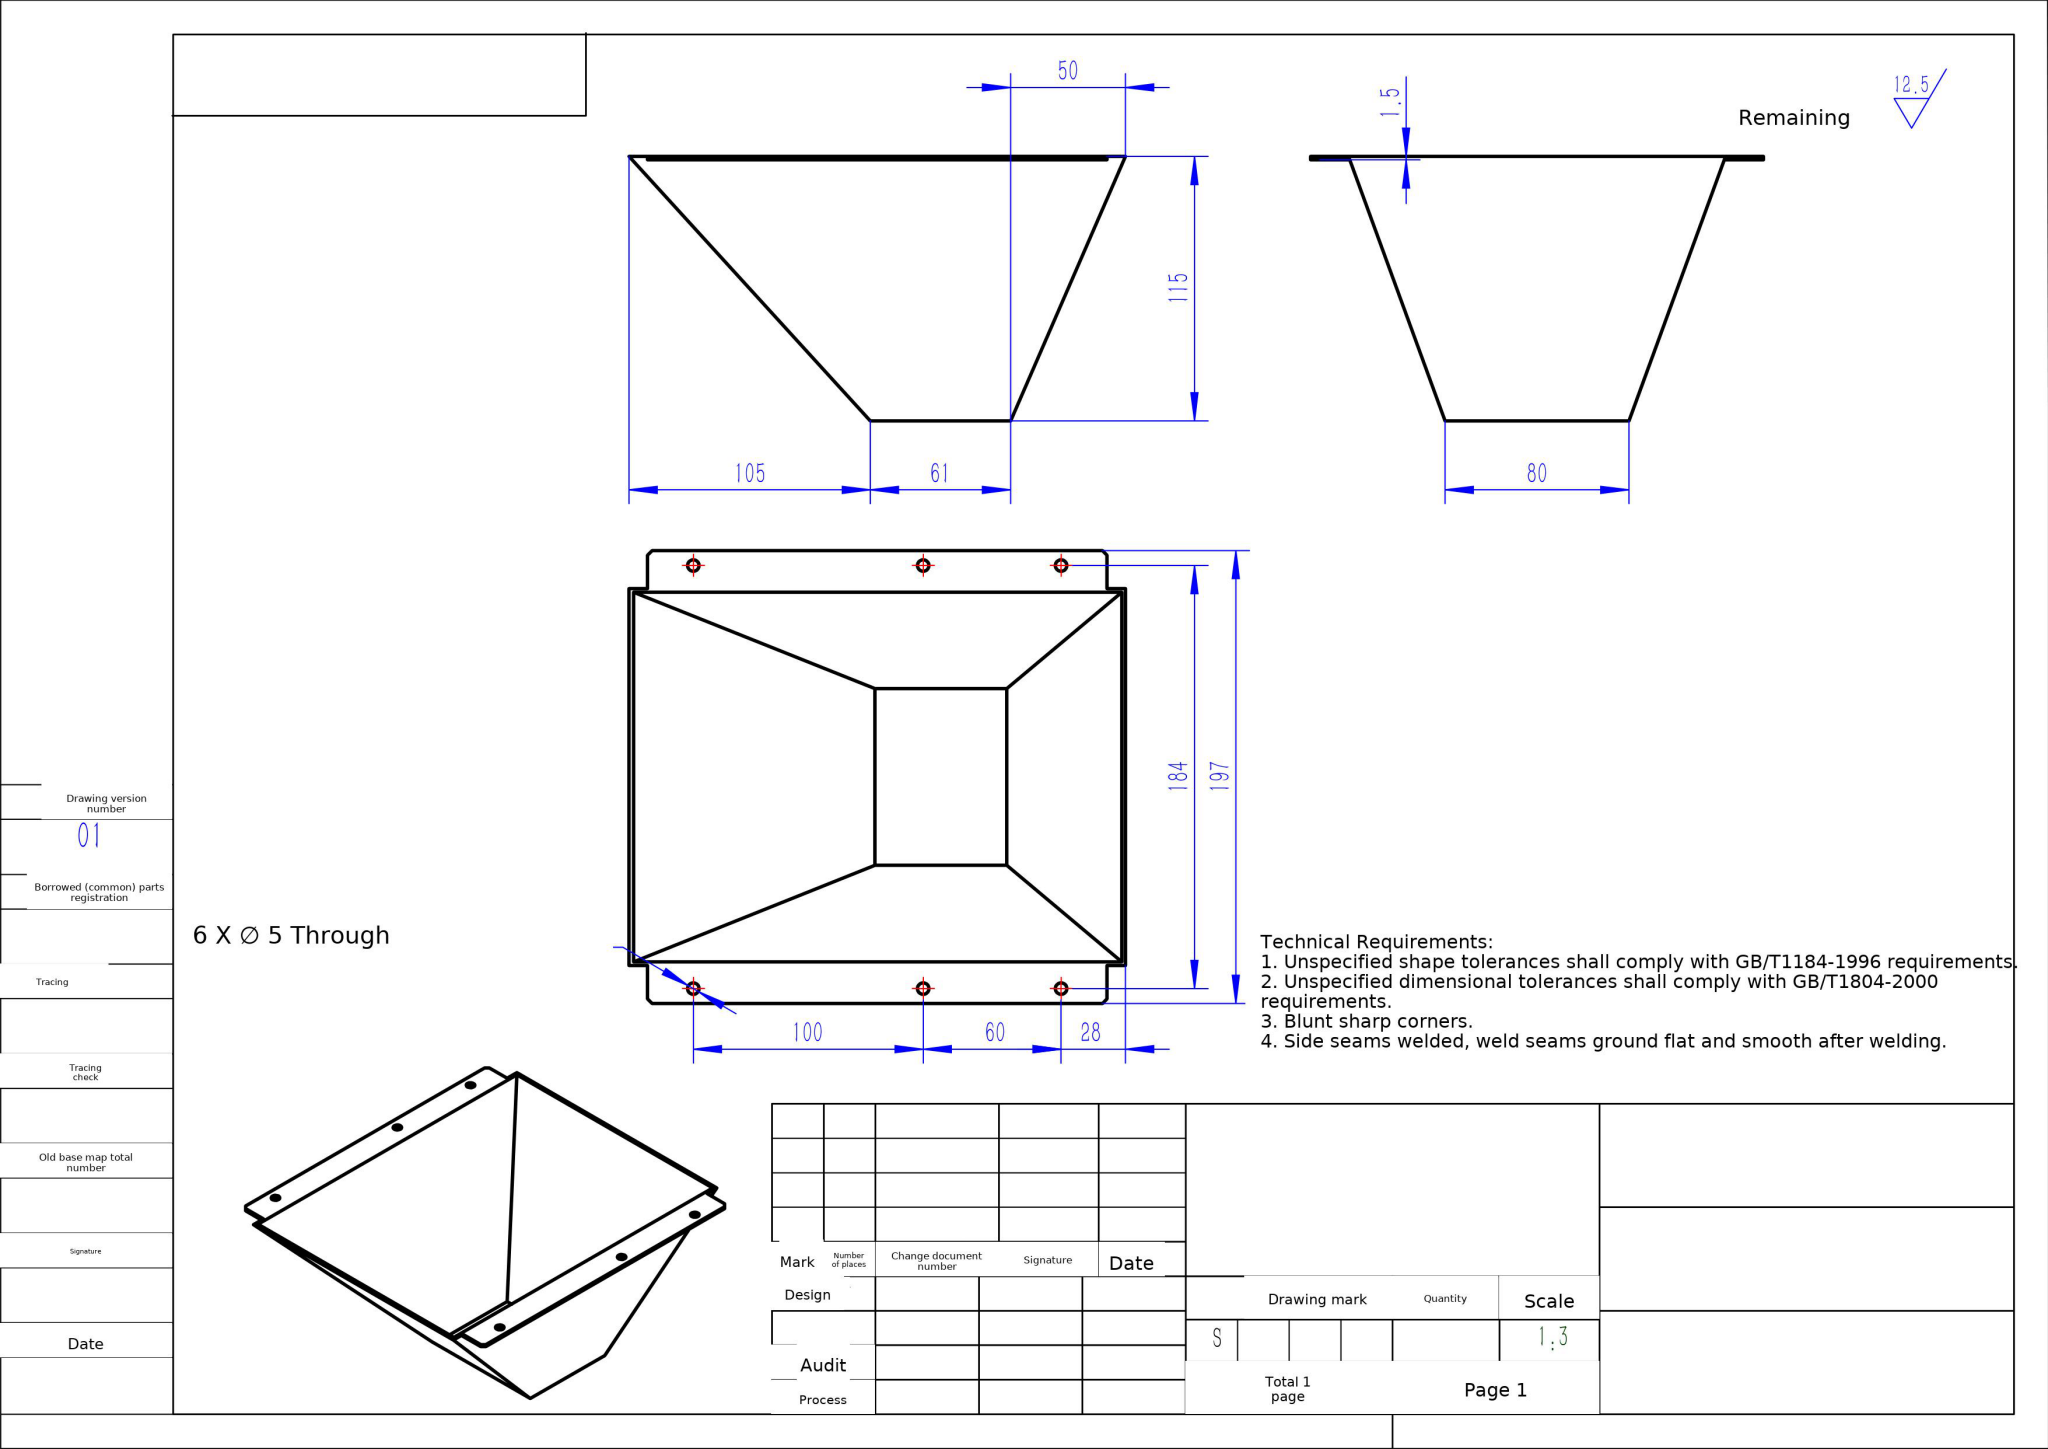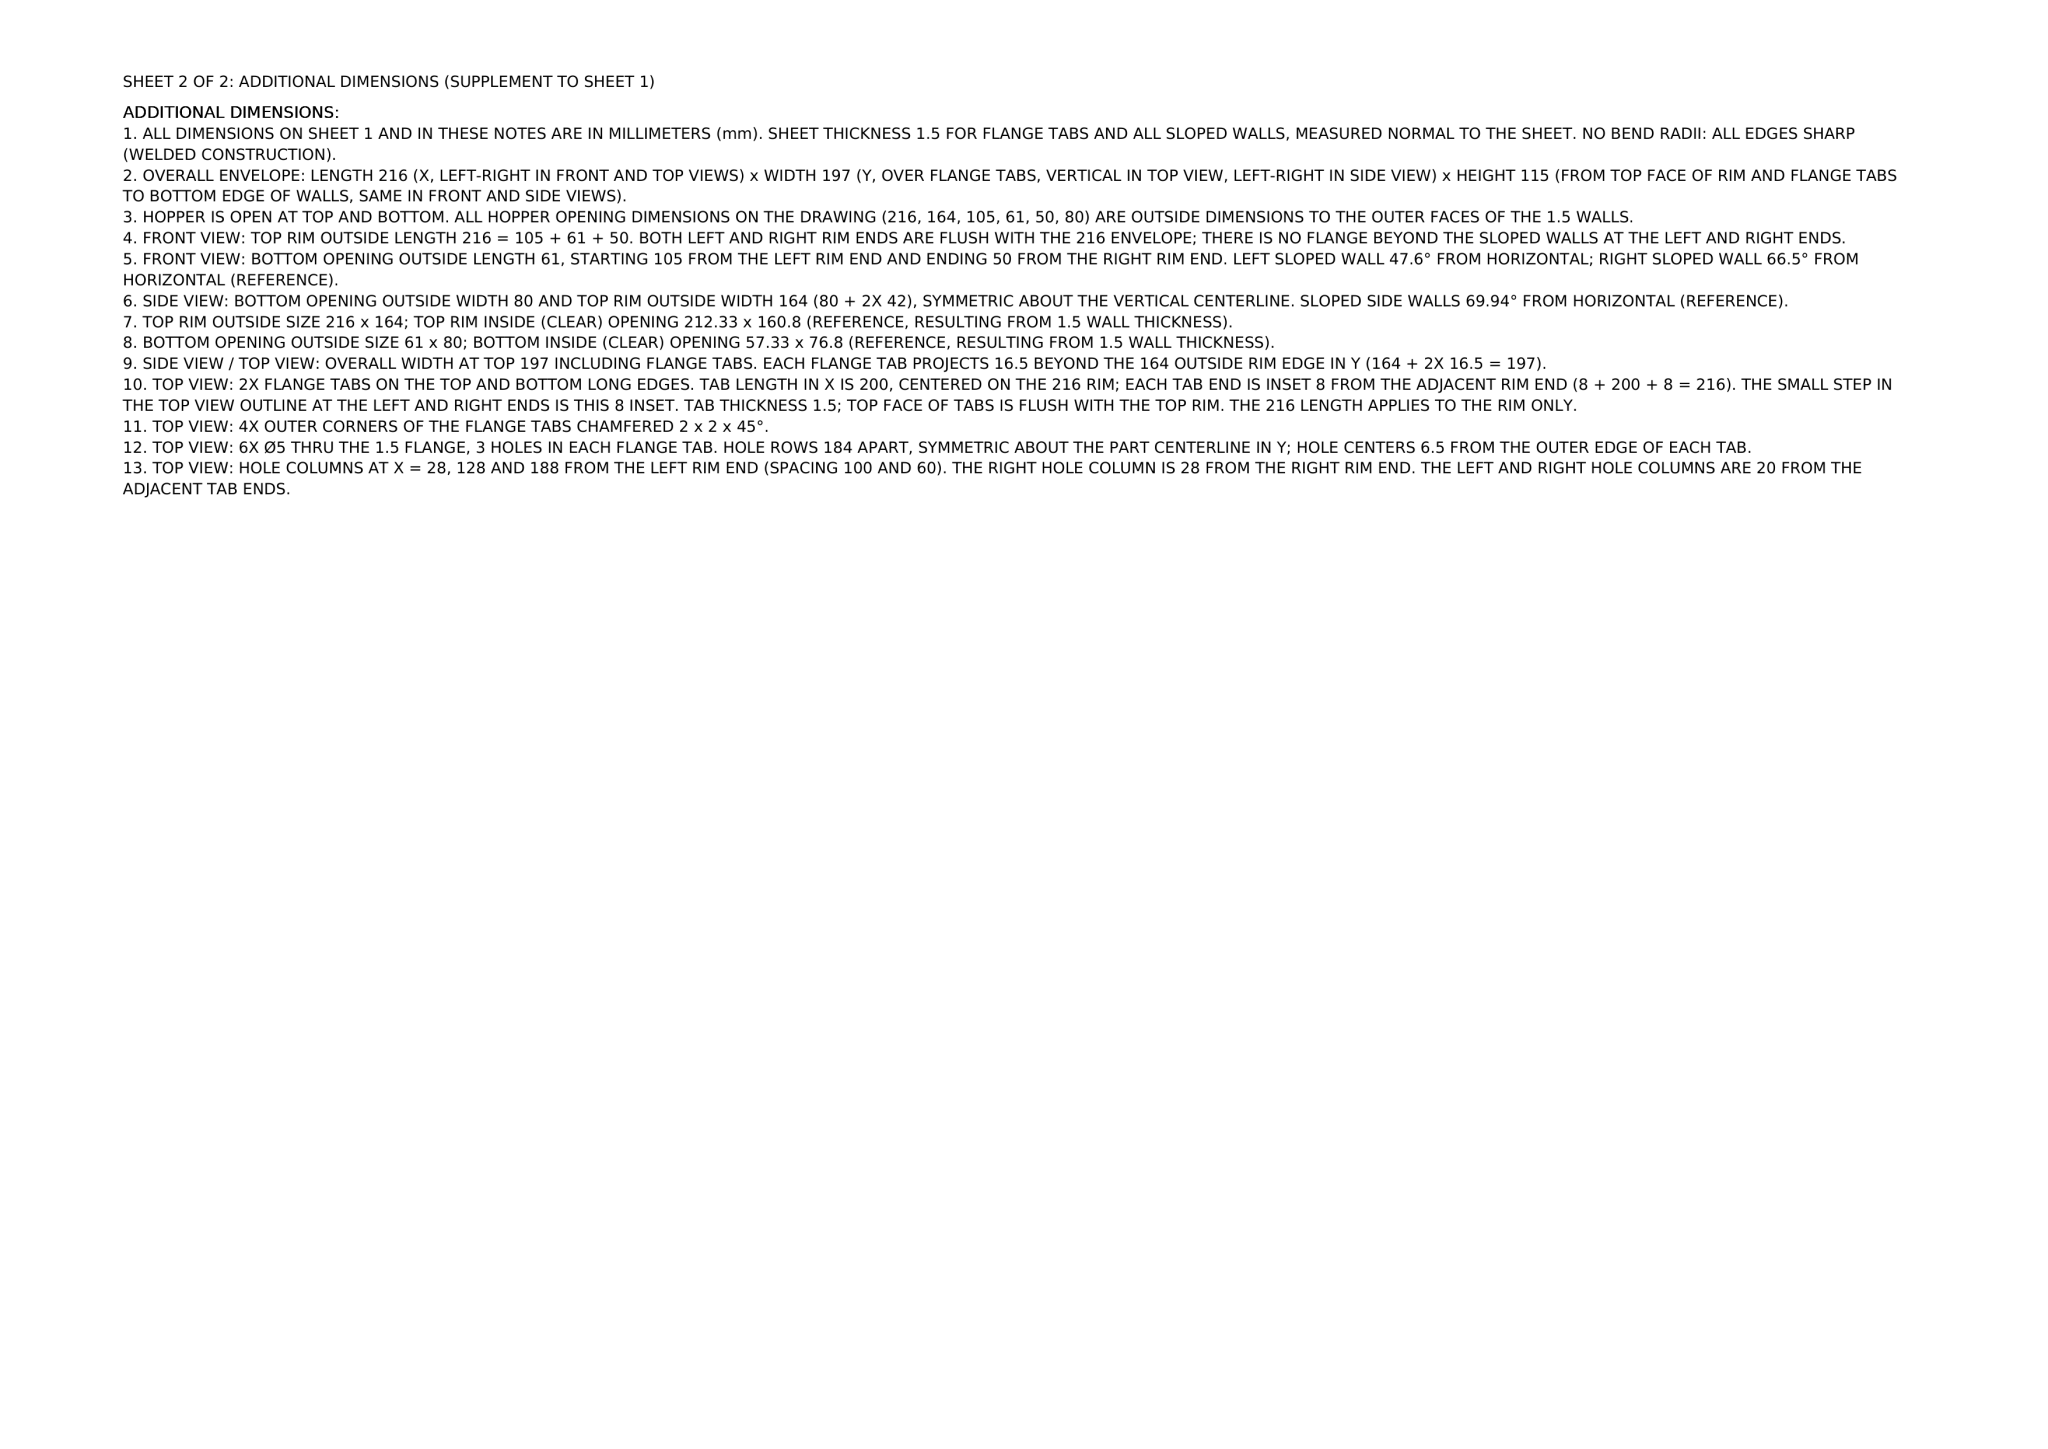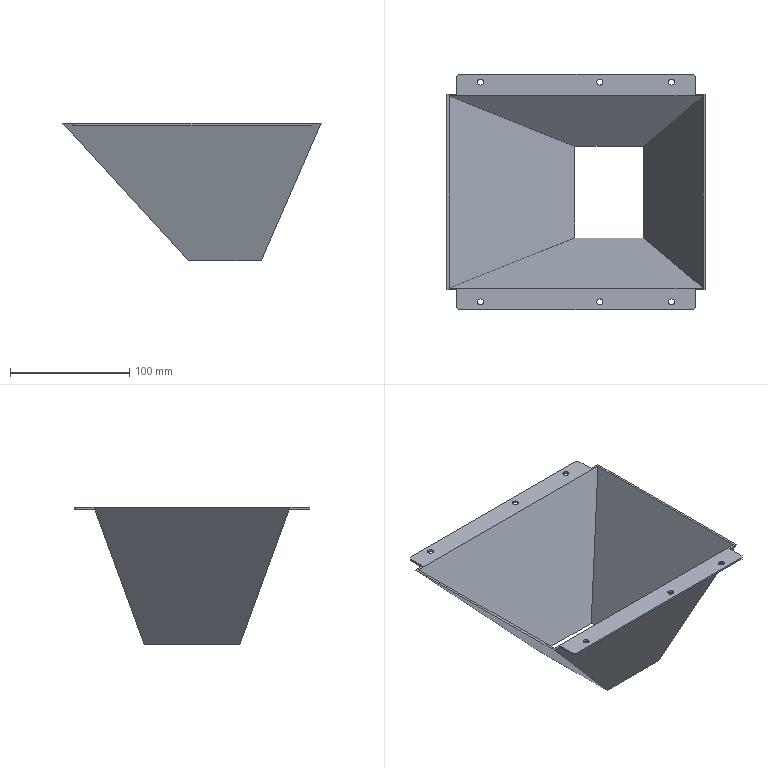Part | NX | mm | 1 solid | 34 faces | box 216 x 197 x 115 mm | volume 110844 mm3 | plane 22 | cylinder 12 | commonest cylinder face diameters 5 x12